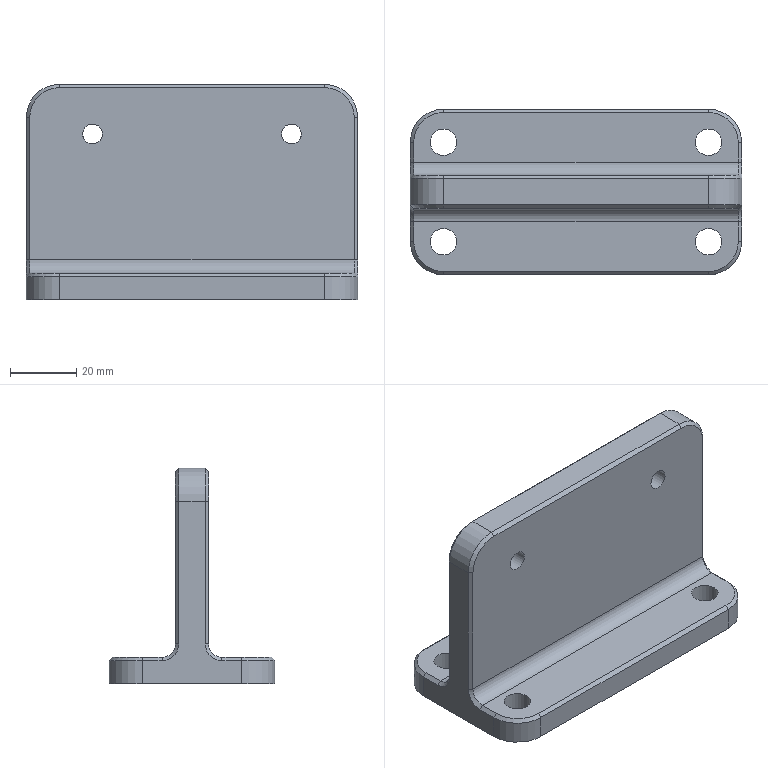Component | NX | BRACKET | 1 solid | 48 faces | volume 94064 mm3 | plane 22 | cylinder 14 | cone 12 | commonest cylinder face diameters 20 x6 8 x6 6 x2